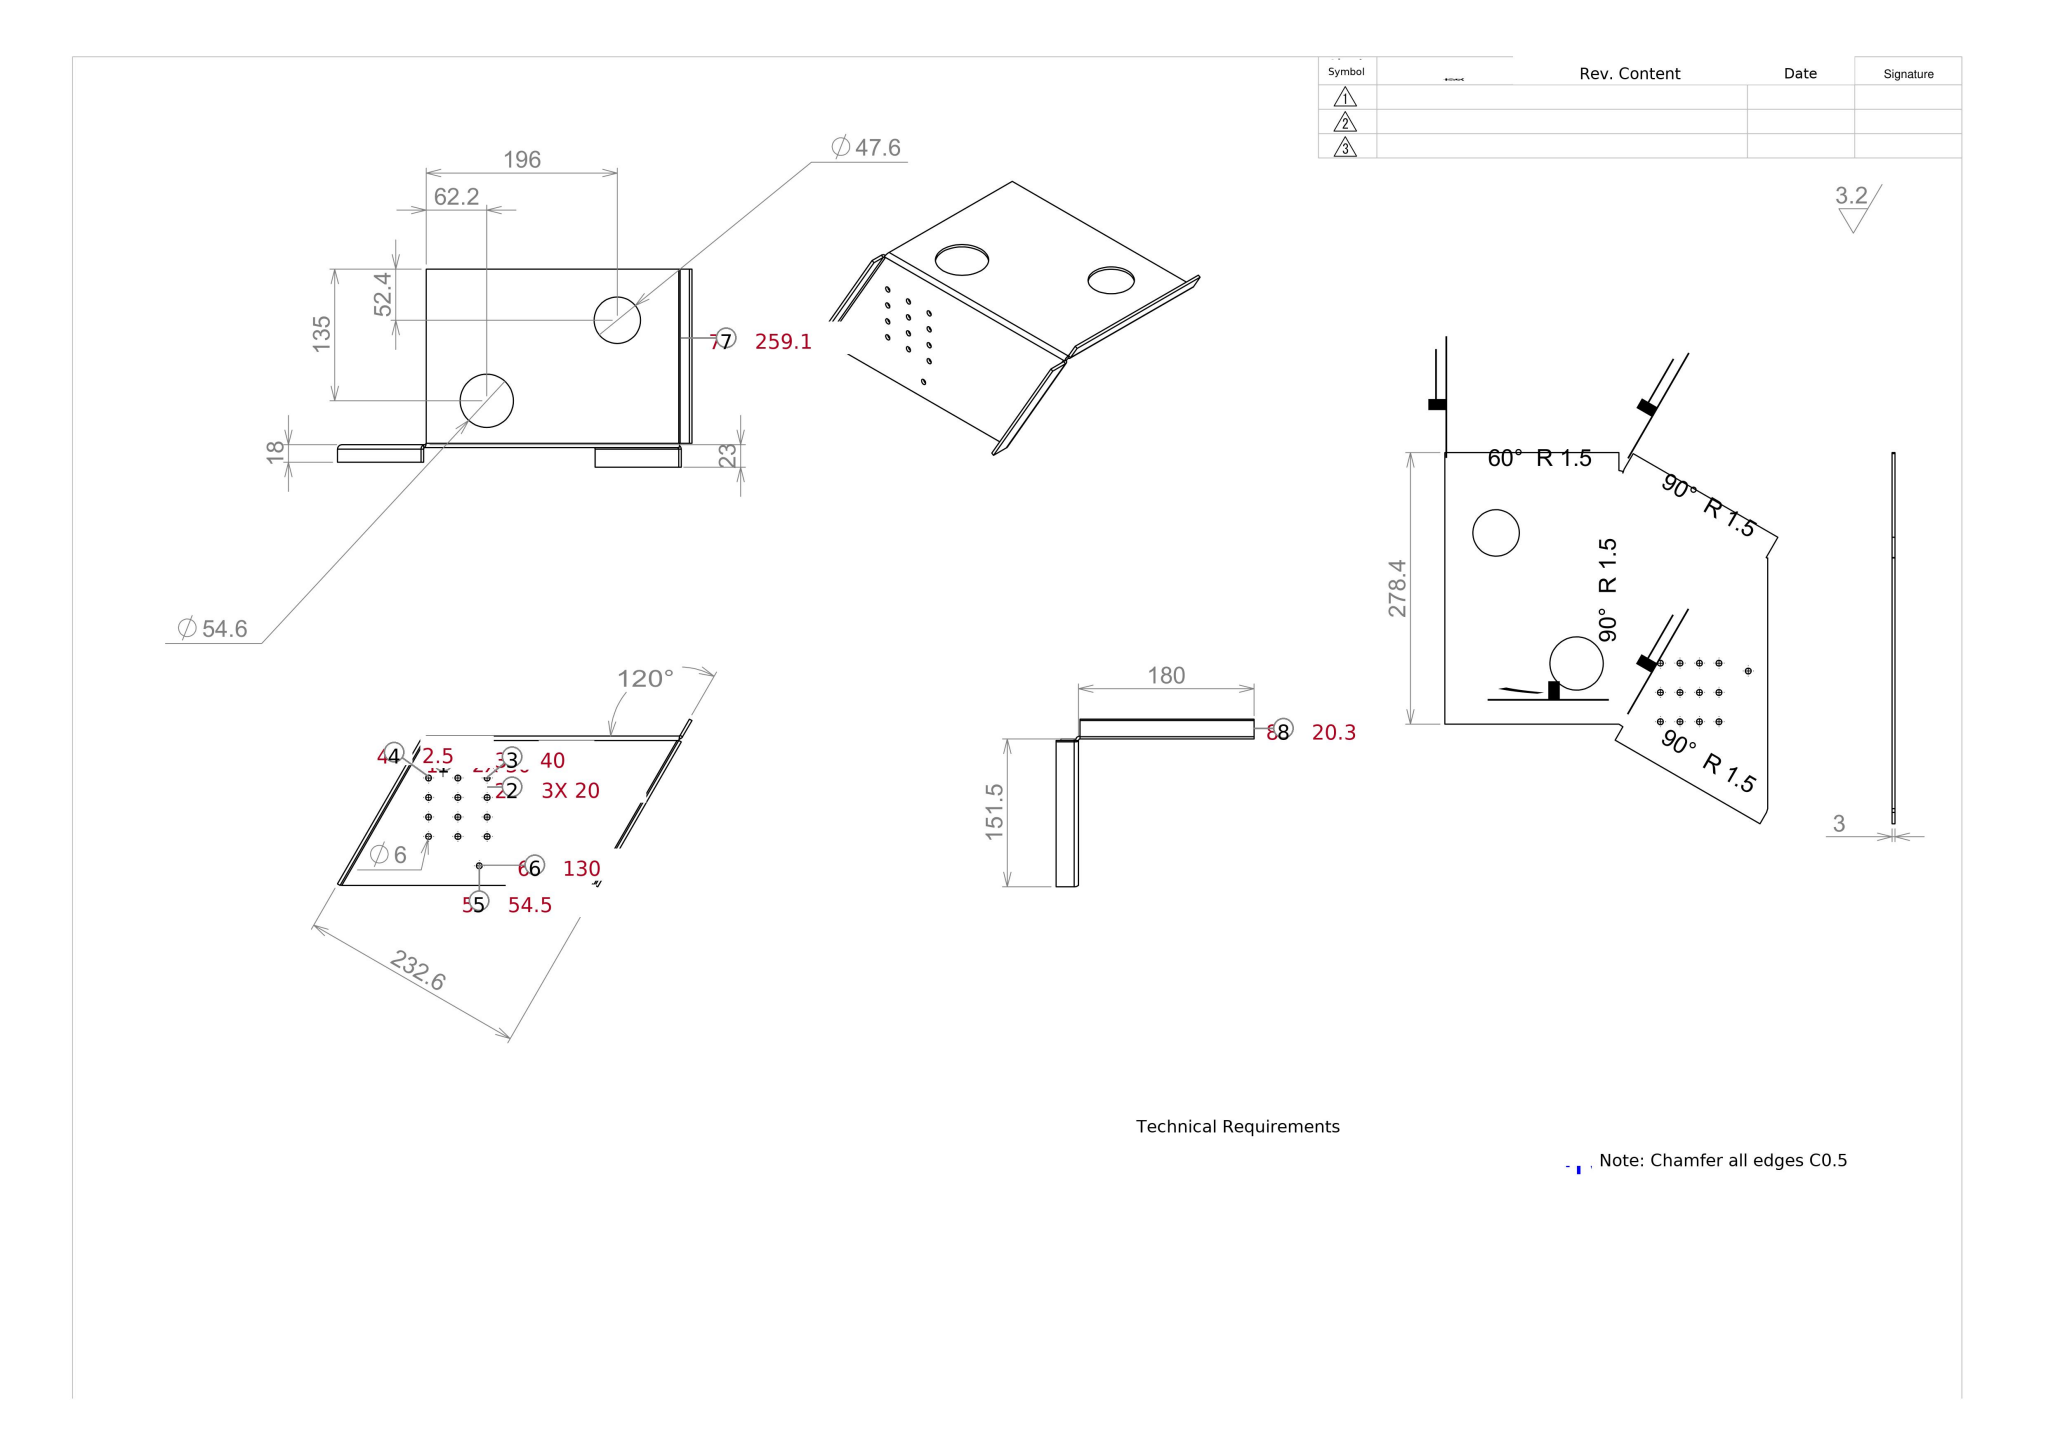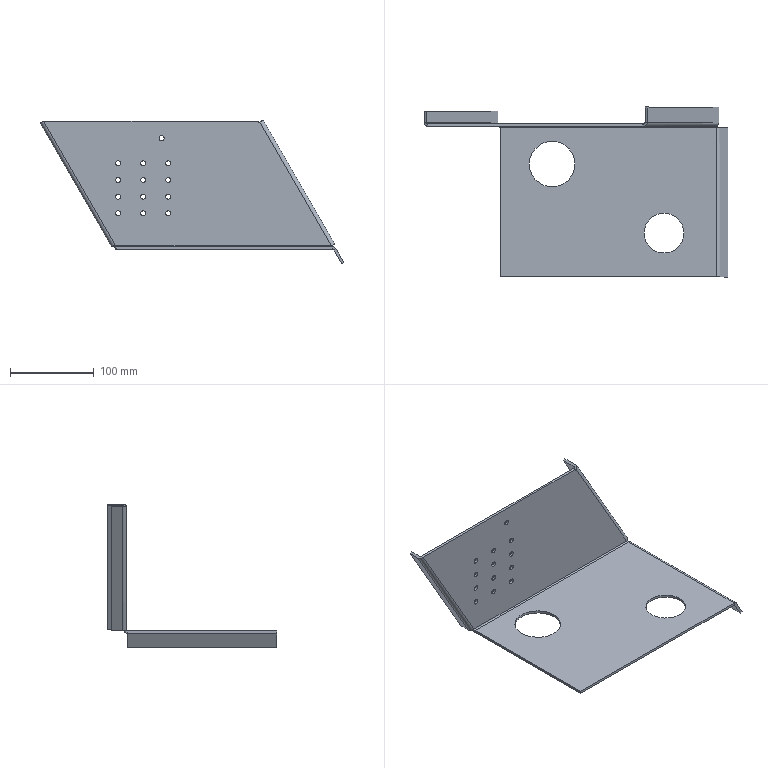Part | SolidWorks | mm | 1 solid | 74 faces | box 363.46 x 203 x 171.82 mm | volume 277192 mm3 | cylinder 38 | plane 32 | spline 4 | commonest cylinder face diameters 6 x26 9 x4 3 x4 54.61 x2 47.623 x2